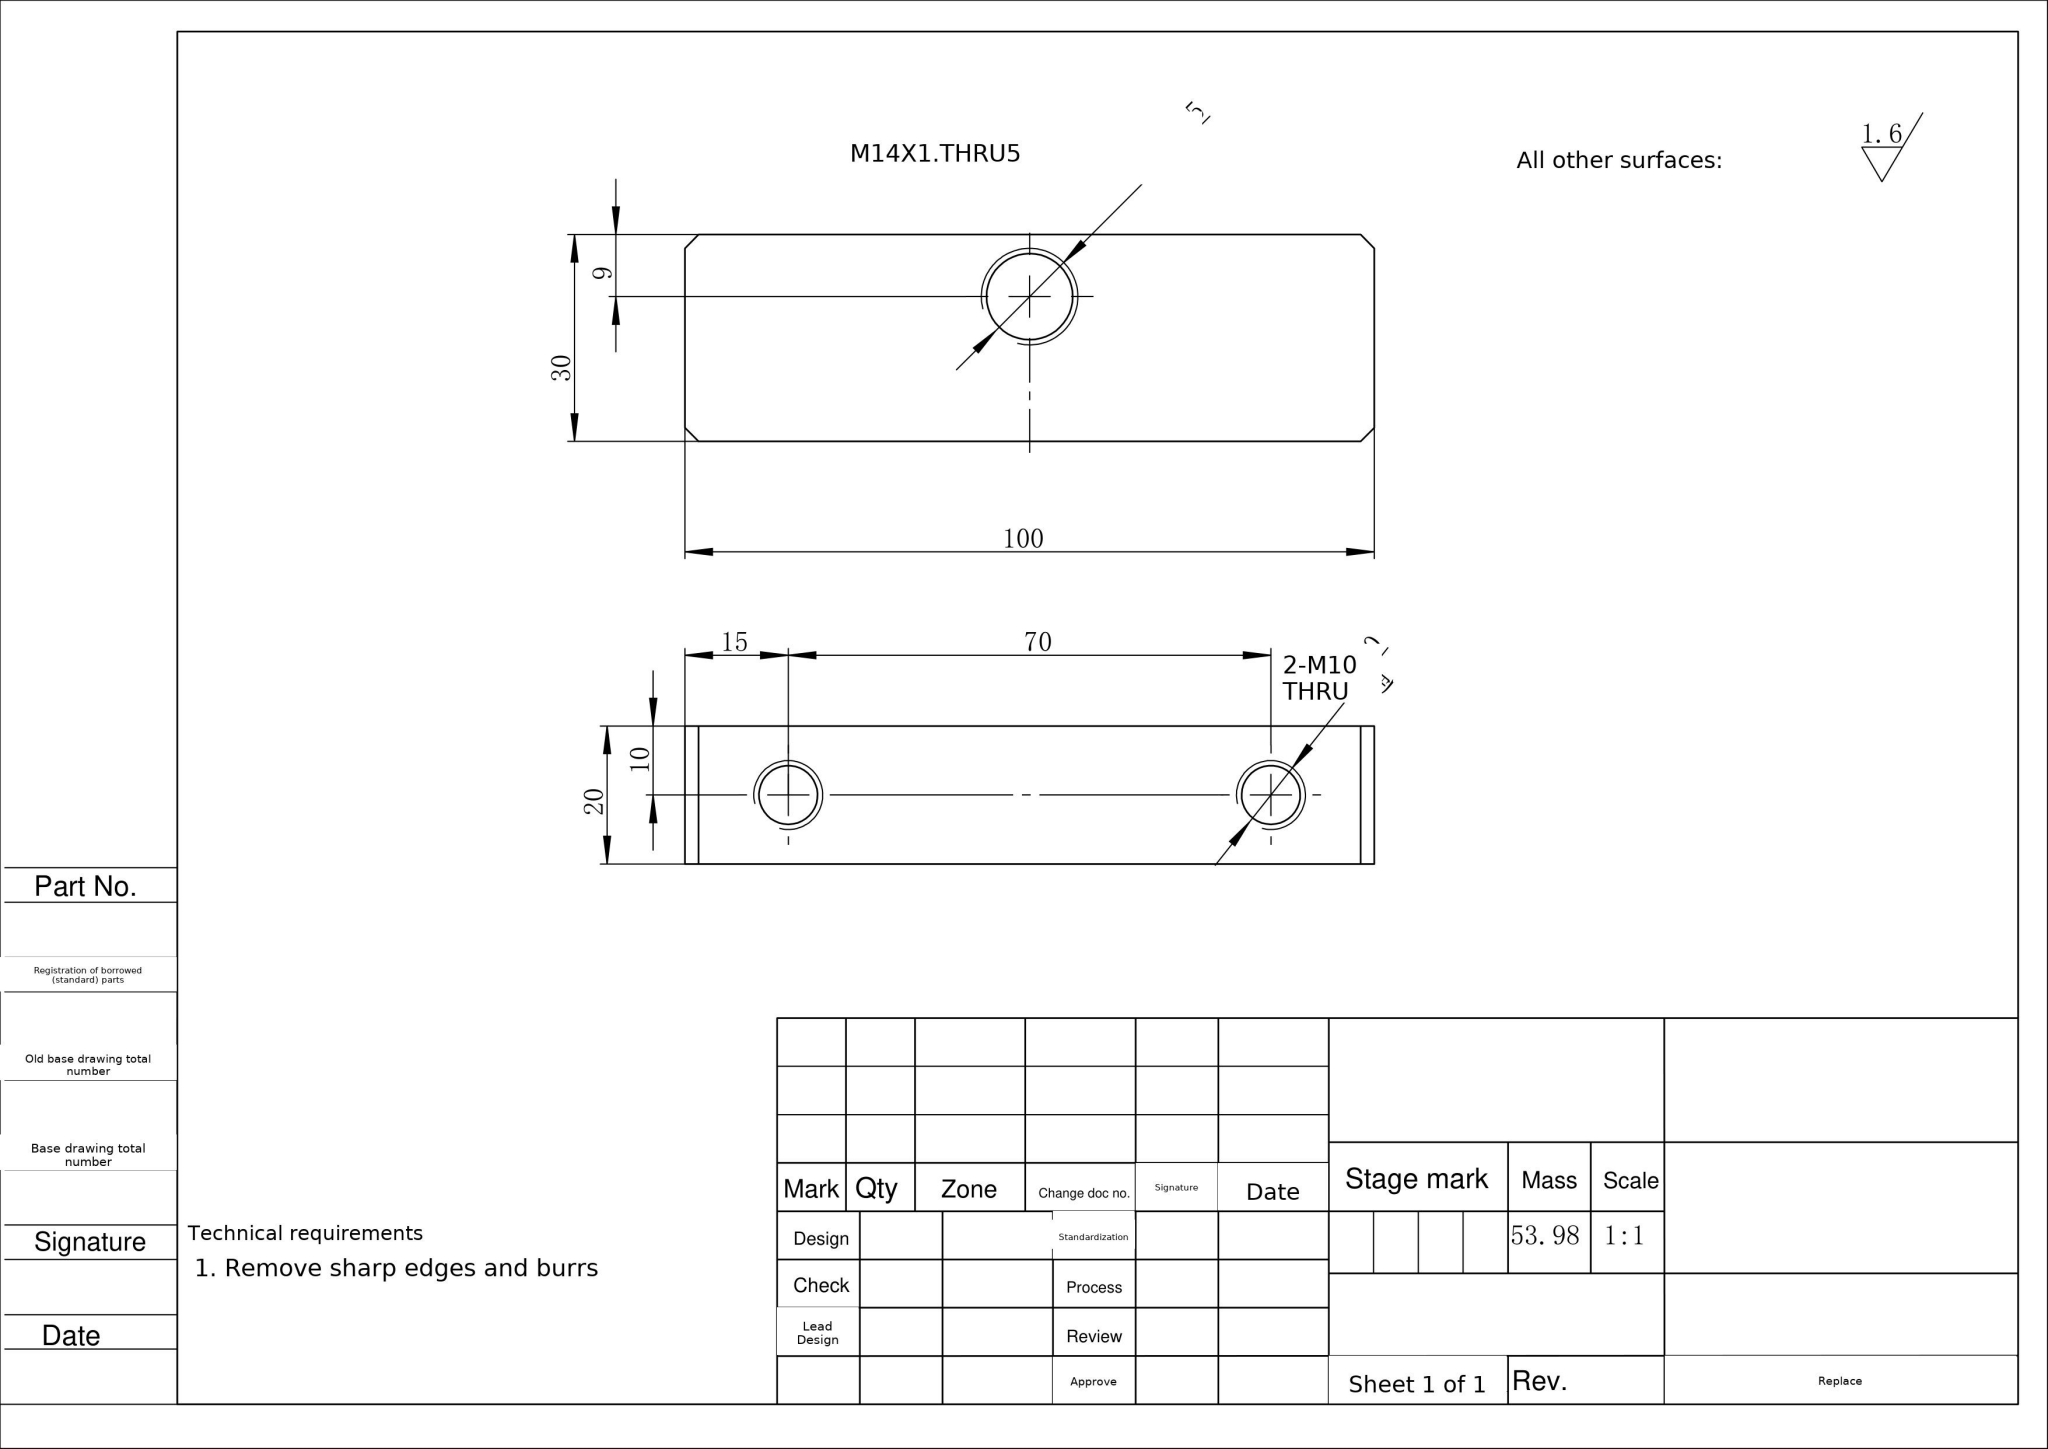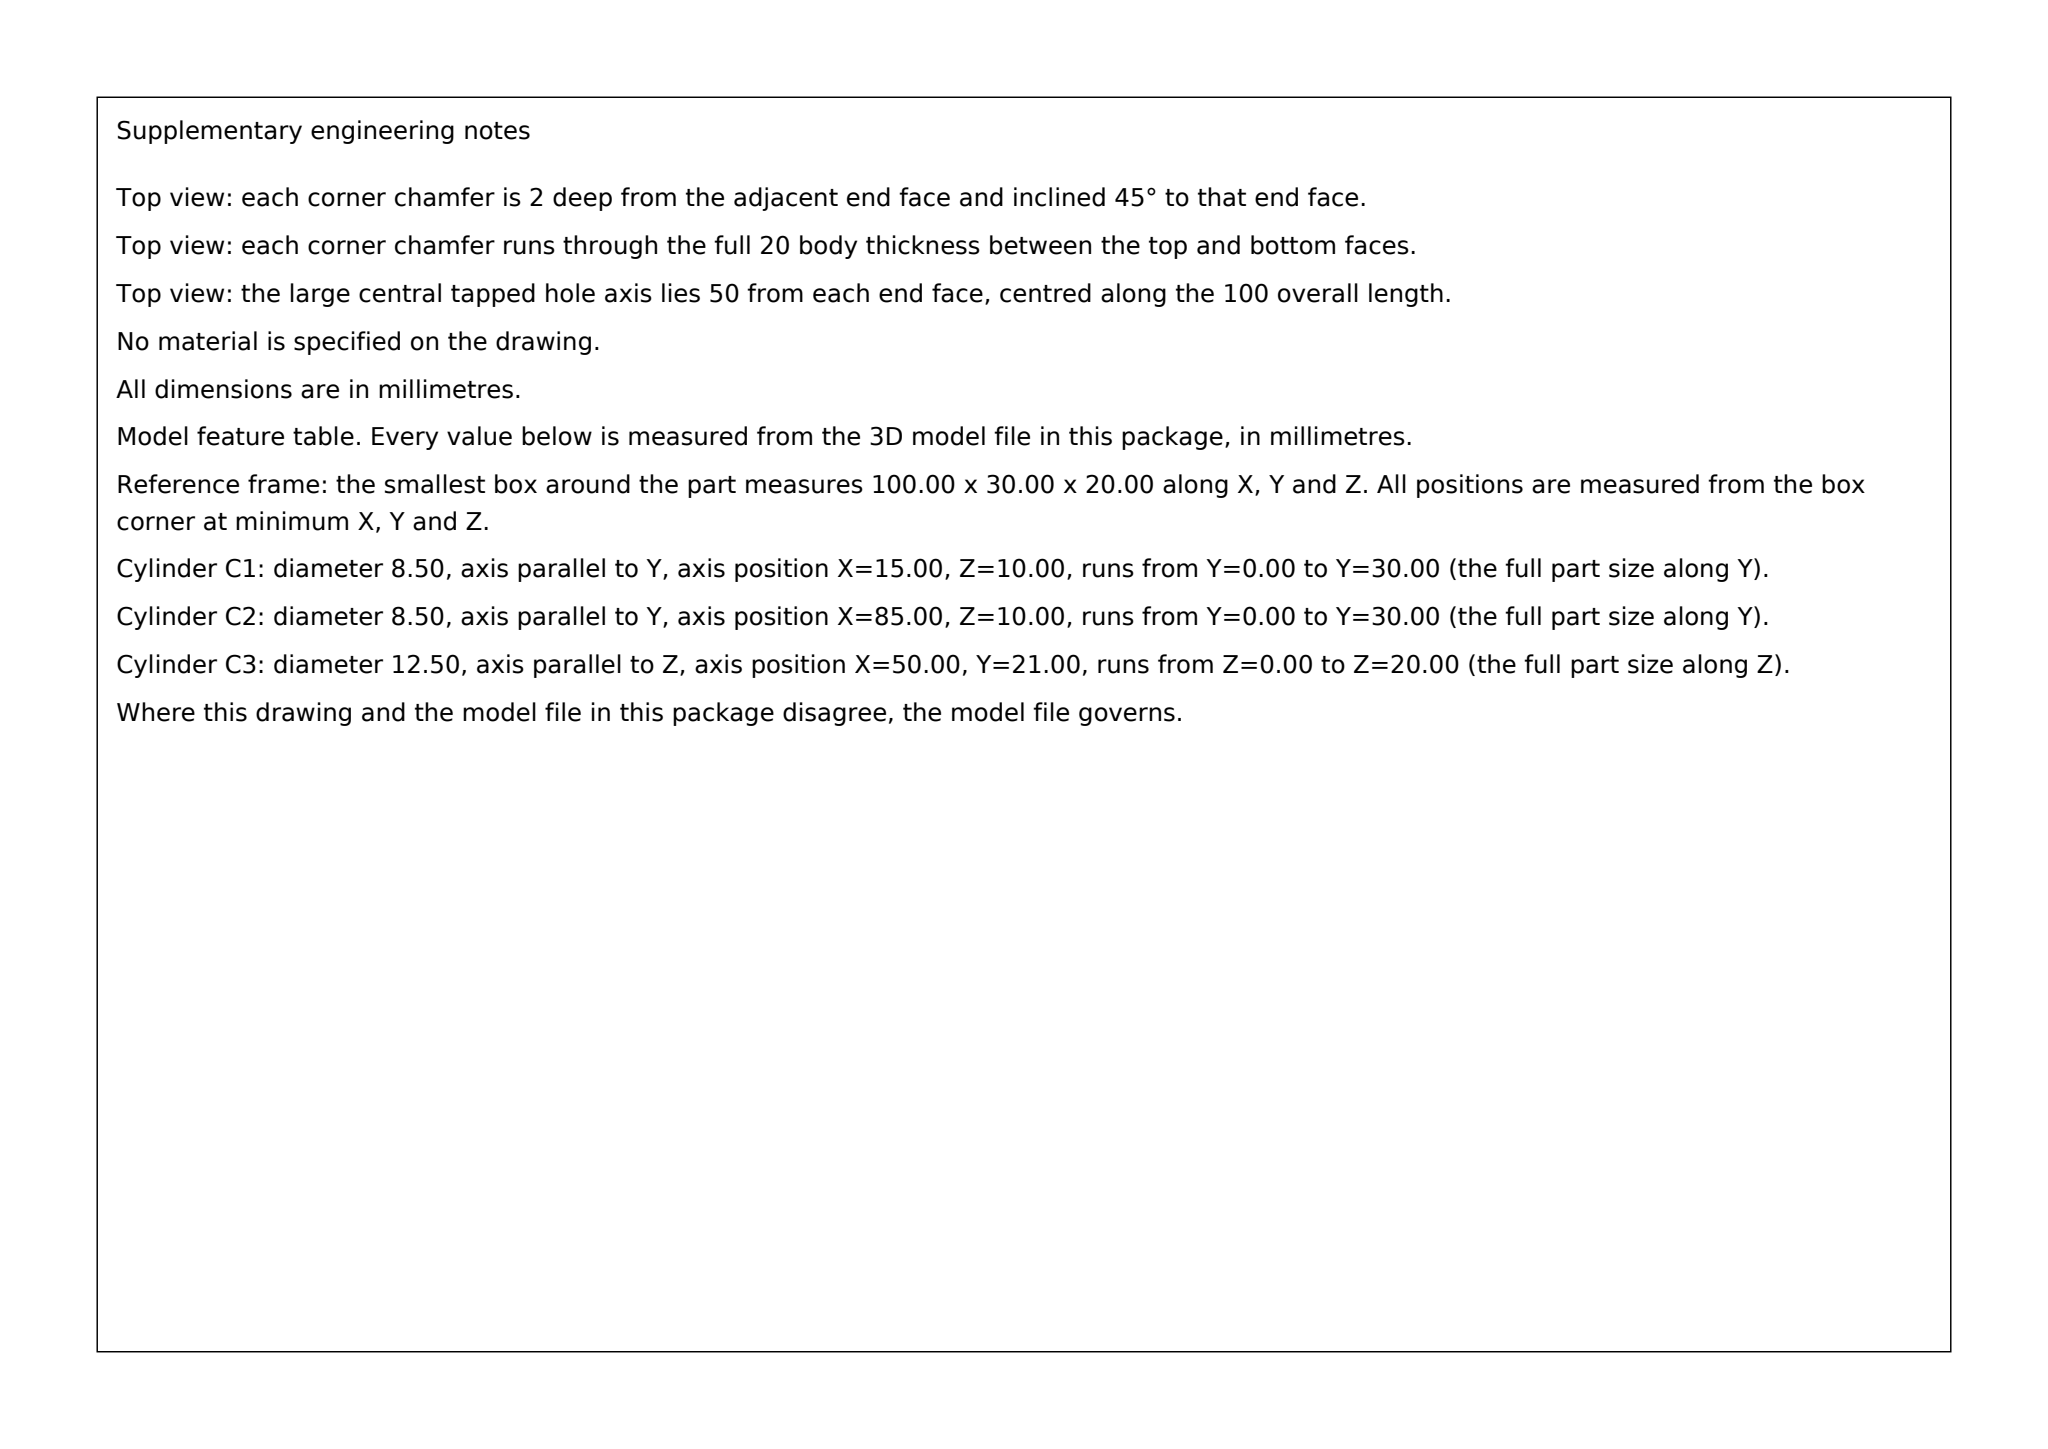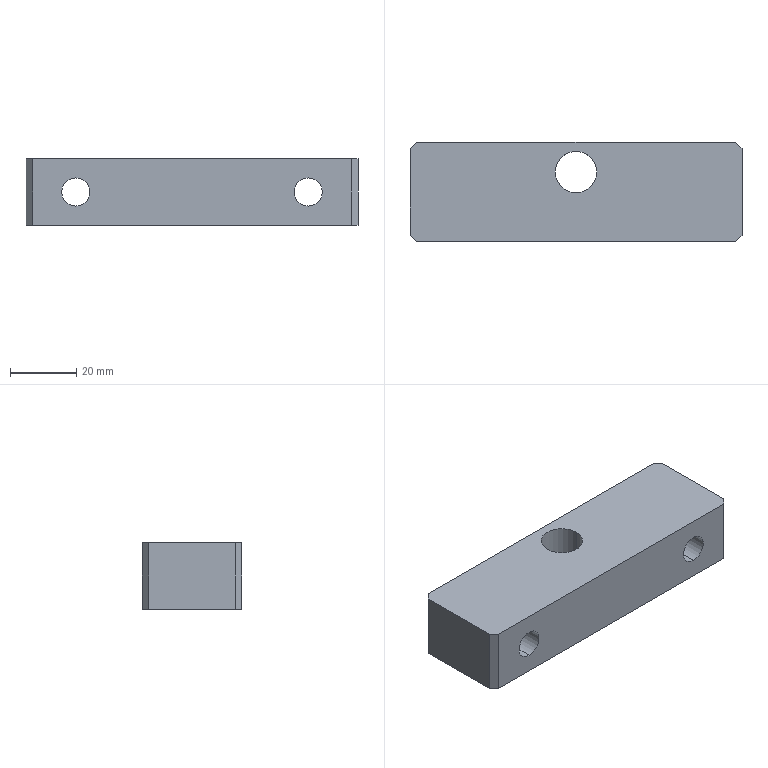Part | SolidWorks | mm | 1 solid | 16 faces | box 100 x 30 x 20 mm | volume 53981 mm3 | plane 10 | cylinder 6 | commonest cylinder face diameters 8.5 x4 12.5 x2
Drawing notes:
M14X1 THRU (THRU 20 THK) - NOT 5 DEEP | from the solid: cylinder dia 12.5, axis z, pos (50,21), length 20 = full 20 thk
M14X1 HOLE CL 50 FROM LEFT END, 9 FROM TOP EDGE | from the solid: cyl axis at x=50 of 100 bbox; y=21 of 30 -> 9 from top face y=30
build123d program:
from build123d import *

# Parameters (mm, degrees)
SKETCH1_W              = 100
SKETCH1_H              = 30
BOSS_EXTRUDE1_DEPTH    = 20
M10_TAPPED_HOLE1_D     = 8.5
M14X1_5_TAPPED_HOLE1_D = 12.5
CHAMFER1_SIZE          = 2


with BuildPart() as part:
    # Sketch1 → Boss-Extrude1 (new body)
    with BuildSketch(Plane.XY):
        Rectangle(SKETCH1_W, SKETCH1_H)
    extrude(amount=BOSS_EXTRUDE1_DEPTH)

    # M10 Tapped Hole1 (through all)
    with Locations(Plane(origin=(0, 15, 0), x_dir=(1, 0, 0), z_dir=(0, 1, 0))):
        with Locations((-35, -10), (35, -10)):
            Hole(M10_TAPPED_HOLE1_D / 2)

    # M14x1.5 Tapped Hole1 (through all)
    with Locations(Plane.XY.offset(20)):
        with Locations((0, 6)):
            Hole(M14X1_5_TAPPED_HOLE1_D / 2)

    # Chamfer1
    chamfer1_edges = [part.edges().sort_by_distance(p)[0] for p in [
        (50, -15, 10),
        (-50, -15, 10),
        (-50, 15, 10),
        (50, 15, 10),
    ]]
    chamfer(chamfer1_edges, length=CHAMFER1_SIZE)


solid = part.part
STEP:
#1=CARTESIAN_POINT('',(6.25,6.,0.));
#2=VERTEX_POINT('',#1);
#3=CARTESIAN_POINT('',(-6.25,6.,0.));
#4=VERTEX_POINT('',#3);
#5=CARTESIAN_POINT('',(0.,6.,0.));
#6=DIRECTION('',(0.,0.,-1.));
#7=DIRECTION('',(-1.,0.,0.));
#8=AXIS2_PLACEMENT_3D('',#5,#6,#7);
#9=CIRCLE('',#8,6.25);
#10=EDGE_CURVE('',#2,#4,#9,.T.);
#11=ORIENTED_EDGE('',*,*,#10,.T.);
#12=CARTESIAN_POINT('',(-6.25,6.,20.));
#13=VERTEX_POINT('',#12);
#14=CARTESIAN_POINT('',(-6.25,6.,20.));
#15=DIRECTION('',(0.,0.,1.));
#16=VECTOR('',#15,1000.);
#17=LINE('',#14,#16);
#18=EDGE_CURVE('',#4,#13,#17,.T.);
#19=ORIENTED_EDGE('',*,*,#18,.T.);
#20=CARTESIAN_POINT('',(6.25,6.,20.));
#21=VERTEX_POINT('',#20);
#22=CARTESIAN_POINT('',(0.,6.,20.));
#23=DIRECTION('',(0.,0.,1.));
#24=DIRECTION('',(1.,0.,0.));
#25=AXIS2_PLACEMENT_3D('',#22,#23,#24);
#26=CIRCLE('',#25,6.25);
#27=EDGE_CURVE('',#13,#21,#26,.T.);
#28=ORIENTED_EDGE('',*,*,#27,.T.);
#29=CARTESIAN_POINT('',(6.25,6.,20.));
#30=DIRECTION('',(0.,0.,1.));
#31=VECTOR('',#30,1000.);
#32=LINE('',#29,#31);
#33=EDGE_CURVE('',#2,#21,#32,.T.);
#34=ORIENTED_EDGE('',*,*,#33,.F.);
#35=EDGE_LOOP('',(#11,#19,#28,#34));
#36=FACE_OUTER_BOUND('',#35,.T.);
#37=CARTESIAN_POINT('',(0.,6.,20.));
#38=DIRECTION('',(0.,0.,1.));
#39=DIRECTION('',(1.,0.,0.));
#40=AXIS2_PLACEMENT_3D('',#37,#38,#39);
#41=CYLINDRICAL_SURFACE('',#40,6.25);
#42=ADVANCED_FACE('',(#36),#41,.F.);
#43=CARTESIAN_POINT('',(-35.,-15.,5.75));
#44=VERTEX_POINT('',#43);
#45=CARTESIAN_POINT('',(-35.,-15.,14.25));
#46=VERTEX_POINT('',#45);
#47=CARTESIAN_POINT('',(-35.,-15.,10.));
#48=DIRECTION('',(0.,1.,0.));
#49=DIRECTION('',(0.,0.,1.));
#50=AXIS2_PLACEMENT_3D('',#47,#48,#49);
#51=CIRCLE('',#50,4.25);
#52=EDGE_CURVE('',#44,#46,#51,.T.);
#53=ORIENTED_EDGE('',*,*,#52,.F.);
#54=CARTESIAN_POINT('',(-35.,15.,5.75));
#55=VERTEX_POINT('',#54);
#56=CARTESIAN_POINT('',(-35.,15.,5.75));
#57=DIRECTION('',(0.,1.,0.));
#58=VECTOR('',#57,1000.);
#59=LINE('',#56,#58);
#60=EDGE_CURVE('',#44,#55,#59,.T.);
#61=ORIENTED_EDGE('',*,*,#60,.T.);
#62=CARTESIAN_POINT('',(-35.,15.,14.25));
#63=VERTEX_POINT('',#62);
#64=CARTESIAN_POINT('',(-35.,15.,10.));
#65=DIRECTION('',(0.,1.,0.));
#66=DIRECTION('',(0.,0.,1.));
#67=AXIS2_PLACEMENT_3D('',#64,#65,#66);
#68=CIRCLE('',#67,4.25);
#69=EDGE_CURVE('',#55,#63,#68,.T.);
#70=ORIENTED_EDGE('',*,*,#69,.T.);
#71=CARTESIAN_POINT('',(-35.,15.,14.25));
#72=DIRECTION('',(0.,1.,0.));
#73=VECTOR('',#72,1000.);
#74=LINE('',#71,#73);
#75=EDGE_CURVE('',#46,#63,#74,.T.);
#76=ORIENTED_EDGE('',*,*,#75,.F.);
#77=EDGE_LOOP('',(#53,#61,#70,#76));
#78=FACE_OUTER_BOUND('',#77,.T.);
#79=CARTESIAN_POINT('',(-35.,15.,10.));
#80=DIRECTION('',(0.,1.,0.));
#81=DIRECTION('',(0.,0.,1.));
#82=AXIS2_PLACEMENT_3D('',#79,#80,#81);
#83=CYLINDRICAL_SURFACE('',#82,4.25);
#84=ADVANCED_FACE('',(#78),#83,.F.);
#85=CARTESIAN_POINT('',(35.,-15.,5.75));
#86=VERTEX_POINT('',#85);
#87=CARTESIAN_POINT('',(35.,-15.,14.25));
#88=VERTEX_POINT('',#87);
#89=CARTESIAN_POINT('',(35.,-15.,10.));
#90=DIRECTION('',(0.,1.,0.));
#91=DIRECTION('',(0.,0.,1.));
#92=AXIS2_PLACEMENT_3D('',#89,#90,#91);
#93=CIRCLE('',#92,4.25);
#94=EDGE_CURVE('',#86,#88,#93,.T.);
#95=ORIENTED_EDGE('',*,*,#94,.F.);
#96=CARTESIAN_POINT('',(35.,15.,5.75));
#97=VERTEX_POINT('',#96);
#98=CARTESIAN_POINT('',(35.,15.,5.75));
#99=DIRECTION('',(0.,1.,0.));
#100=VECTOR('',#99,1000.);
#101=LINE('',#98,#100);
#102=EDGE_CURVE('',#86,#97,#101,.T.);
#103=ORIENTED_EDGE('',*,*,#102,.T.);
#104=CARTESIAN_POINT('',(35.,15.,14.25));
#105=VERTEX_POINT('',#104);
#106=CARTESIAN_POINT('',(35.,15.,10.));
#107=DIRECTION('',(0.,1.,0.));
#108=DIRECTION('',(0.,0.,1.));
#109=AXIS2_PLACEMENT_3D('',#106,#107,#108);
#110=CIRCLE('',#109,4.25);
#111=EDGE_CURVE('',#97,#105,#110,.T.);
#112=ORIENTED_EDGE('',*,*,#111,.T.);
#113=CARTESIAN_POINT('',(35.,15.,14.25));
#114=DIRECTION('',(0.,1.,0.));
#115=VECTOR('',#114,1000.);
#116=LINE('',#113,#115);
#117=EDGE_CURVE('',#88,#105,#116,.T.);
#118=ORIENTED_EDGE('',*,*,#117,.F.);
#119=EDGE_LOOP('',(#95,#103,#112,#118));
#120=FACE_OUTER_BOUND('',#119,.T.);
#121=CARTESIAN_POINT('',(35.,15.,10.));
#122=DIRECTION('',(0.,1.,0.));
#123=DIRECTION('',(0.,0.,1.));
#124=AXIS2_PLACEMENT_3D('',#121,#122,#123);
#125=CYLINDRICAL_SURFACE('',#124,4.25);
#126=ADVANCED_FACE('',(#120),#125,.F.);
#127=CARTESIAN_POINT('',(48.,15.,0.));
#128=VERTEX_POINT('',#127);
#129=CARTESIAN_POINT('',(-48.,15.,0.));
#130=VERTEX_POINT('',#129);
#131=CARTESIAN_POINT('',(-50.,15.,0.));
#132=DIRECTION('',(-1.,0.,0.));
#133=VECTOR('',#132,1000.);
#134=LINE('',#131,#133);
#135=EDGE_CURVE('',#128,#130,#134,.T.);
#136=ORIENTED_EDGE('',*,*,#135,.T.);
#137=CARTESIAN_POINT('',(-48.,15.,20.));
#138=VERTEX_POINT('',#137);
#139=CARTESIAN_POINT('',(-48.,15.,20.));
#140=DIRECTION('',(0.,0.,1.));
#141=VECTOR('',#140,1000.);
#142=LINE('',#139,#141);
#143=EDGE_CURVE('',#130,#138,#142,.T.);
#144=ORIENTED_EDGE('',*,*,#143,.T.);
#145=CARTESIAN_POINT('',(48.,15.,20.));
#146=VERTEX_POINT('',#145);
#147=CARTESIAN_POINT('',(-50.,15.,20.));
#148=DIRECTION('',(-1.,0.,0.));
#149=VECTOR('',#148,1000.);
#150=LINE('',#147,#149);
#151=EDGE_CURVE('',#146,#138,#150,.T.);
#152=ORIENTED_EDGE('',*,*,#151,.F.);
#153=CARTESIAN_POINT('',(48.,15.,20.));
#154=DIRECTION('',(0.,0.,-1.));
#155=VECTOR('',#154,1000.);
#156=LINE('',#153,#155);
#157=EDGE_CURVE('',#146,#128,#156,.T.);
#158=ORIENTED_EDGE('',*,*,#157,.T.);
#159=EDGE_LOOP('',(#136,#144,#152,#158));
#160=FACE_OUTER_BOUND('',#159,.T.);
#161=CARTESIAN_POINT('',(35.,15.,10.));
#162=DIRECTION('',(0.,1.,0.));
#163=DIRECTION('',(0.,0.,1.));
#164=AXIS2_PLACEMENT_3D('',#161,#162,#163);
#165=CIRCLE('',#164,4.25);
#166=EDGE_CURVE('',#105,#97,#165,.T.);
#167=ORIENTED_EDGE('',*,*,#166,.F.);
#168=ORIENTED_EDGE('',*,*,#111,.F.);
#169=EDGE_LOOP('',(#167,#168));
#170=FACE_BOUND('',#169,.T.);
#171=CARTESIAN_POINT('',(-35.,15.,10.));
#172=DIRECTION('',(0.,1.,0.));
#173=DIRECTION('',(0.,0.,1.));
#174=AXIS2_PLACEMENT_3D('',#171,#172,#173);
#175=CIRCLE('',#174,4.25);
#176=EDGE_CURVE('',#63,#55,#175,.T.);
#177=ORIENTED_EDGE('',*,*,#176,.F.);
#178=ORIENTED_EDGE('',*,*,#69,.F.);
#179=EDGE_LOOP('',(#177,#178));
#180=FACE_BOUND('',#179,.T.);
#181=CARTESIAN_POINT('',(-50.,15.,20.));
#182=DIRECTION('',(0.,-1.,0.));
#183=DIRECTION('',(0.,0.,-1.));
#184=AXIS2_PLACEMENT_3D('',#181,#182,#183);
#185=PLANE('',#184);
#186=ADVANCED_FACE('',(#160,#170,#180),#185,.F.);
#187=CARTESIAN_POINT('',(50.,-13.,0.));
#188=VERTEX_POINT('',#187);
#189=CARTESIAN_POINT('',(50.,13.,0.));
#190=VERTEX_POINT('',#189);
#191=CARTESIAN_POINT('',(50.,-15.,0.));
#192=DIRECTION('',(0.,1.,0.));
#193=VECTOR('',#192,1000.);
#194=LINE('',#191,#193);
#195=EDGE_CURVE('',#188,#190,#194,.T.);
#196=ORIENTED_EDGE('',*,*,#195,.T.);
#197=CARTESIAN_POINT('',(50.,13.,20.));
#198=VERTEX_POINT('',#197);
#199=CARTESIAN_POINT('',(50.,13.,20.));
#200=DIRECTION('',(0.,0.,1.));
#201=VECTOR('',#200,1000.);
#202=LINE('',#199,#201);
#203=EDGE_CURVE('',#190,#198,#202,.T.);
#204=ORIENTED_EDGE('',*,*,#203,.T.);
#205=CARTESIAN_POINT('',(50.,-13.,20.));
#206=VERTEX_POINT('',#205);
#207=CARTESIAN_POINT('',(50.,-15.,20.));
#208=DIRECTION('',(0.,1.,0.));
#209=VECTOR('',#208,1000.);
#210=LINE('',#207,#209);
#211=EDGE_CURVE('',#206,#198,#210,.T.);
#212=ORIENTED_EDGE('',*,*,#211,.F.);
#213=CARTESIAN_POINT('',(50.,-13.,20.));
#214=DIRECTION('',(0.,0.,-1.));
#215=VECTOR('',#214,1000.);
#216=LINE('',#213,#215);
#217=EDGE_CURVE('',#206,#188,#216,.T.);
#218=ORIENTED_EDGE('',*,*,#217,.T.);
#219=EDGE_LOOP('',(#196,#204,#212,#218));
#220=FACE_OUTER_BOUND('',#219,.T.);
#221=CARTESIAN_POINT('',(50.,-15.,20.));
#222=DIRECTION('',(-1.,0.,0.));
#223=DIRECTION('',(0.,0.,1.));
#224=AXIS2_PLACEMENT_3D('',#221,#222,#223);
#225=PLANE('',#224);
#226=ADVANCED_FACE('',(#220),#225,.F.);
#227=CARTESIAN_POINT('',(-50.,13.,0.));
#228=VERTEX_POINT('',#227);
#229=CARTESIAN_POINT('',(-50.,-13.,0.));
#230=VERTEX_POINT('',#229);
#231=CARTESIAN_POINT('',(-50.,-15.,0.));
#232=DIRECTION('',(0.,-1.,0.));
#233=VECTOR('',#232,1000.);
#234=LINE('',#231,#233);
#235=EDGE_CURVE('',#228,#230,#234,.T.);
#236=ORIENTED_EDGE('',*,*,#235,.T.);
#237=CARTESIAN_POINT('',(-50.,-13.,20.));
#238=VERTEX_POINT('',#237);
#239=CARTESIAN_POINT('',(-50.,-13.,20.));
#240=DIRECTION('',(0.,0.,1.));
#241=VECTOR('',#240,1000.);
#242=LINE('',#239,#241);
#243=EDGE_CURVE('',#230,#238,#242,.T.);
#244=ORIENTED_EDGE('',*,*,#243,.T.);
#245=CARTESIAN_POINT('',(-50.,13.,20.));
#246=VERTEX_POINT('',#245);
#247=CARTESIAN_POINT('',(-50.,-15.,20.));
#248=DIRECTION('',(0.,-1.,0.));
#249=VECTOR('',#248,1000.);
#250=LINE('',#247,#249);
#251=EDGE_CURVE('',#246,#238,#250,.T.);
#252=ORIENTED_EDGE('',*,*,#251,.F.);
#253=CARTESIAN_POINT('',(-50.,13.,20.));
#254=DIRECTION('',(0.,0.,-1.));
#255=VECTOR('',#254,1000.);
#256=LINE('',#253,#255);
#257=EDGE_CURVE('',#246,#228,#256,.T.);
#258=ORIENTED_EDGE('',*,*,#257,.T.);
#259=EDGE_LOOP('',(#236,#244,#252,#258));
#260=FACE_OUTER_BOUND('',#259,.T.);
#261=CARTESIAN_POINT('',(-50.,-15.,20.));
#262=DIRECTION('',(1.,0.,0.));
#263=DIRECTION('',(0.,0.,-1.));
#264=AXIS2_PLACEMENT_3D('',#261,#262,#263);
#265=PLANE('',#264);
#266=ADVANCED_FACE('',(#260),#265,.F.);
#267=CARTESIAN_POINT('',(-35.,-15.,10.));
#268=DIRECTION('',(0.,1.,0.));
#269=DIRECTION('',(0.,0.,1.));
#270=AXIS2_PLACEMENT_3D('',#267,#268,#269);
#271=CIRCLE('',#270,4.25);
#272=EDGE_CURVE('',#46,#44,#271,.T.);
#273=ORIENTED_EDGE('',*,*,#272,.T.);
#274=ORIENTED_EDGE('',*,*,#52,.T.);
#275=EDGE_LOOP('',(#273,#274));
#276=FACE_BOUND('',#275,.T.);
#277=CARTESIAN_POINT('',(35.,-15.,10.));
#278=DIRECTION('',(0.,1.,0.));
#279=DIRECTION('',(0.,0.,1.));
#280=AXIS2_PLACEMENT_3D('',#277,#278,#279);
#281=CIRCLE('',#280,4.25);
#282=EDGE_CURVE('',#88,#86,#281,.T.);
#283=ORIENTED_EDGE('',*,*,#282,.T.);
#284=ORIENTED_EDGE('',*,*,#94,.T.);
#285=EDGE_LOOP('',(#283,#284));
#286=FACE_BOUND('',#285,.T.);
#287=CARTESIAN_POINT('',(-48.,-15.,20.));
#288=VERTEX_POINT('',#287);
#289=CARTESIAN_POINT('',(48.,-15.,20.));
#290=VERTEX_POINT('',#289);
#291=CARTESIAN_POINT('',(-50.,-15.,20.));
#292=DIRECTION('',(1.,0.,0.));
#293=VECTOR('',#292,1000.);
#294=LINE('',#291,#293);
#295=EDGE_CURVE('',#288,#290,#294,.T.);
#296=ORIENTED_EDGE('',*,*,#295,.F.);
#297=CARTESIAN_POINT('',(-48.,-15.,0.));
#298=VERTEX_POINT('',#297);
#299=CARTESIAN_POINT('',(-48.,-15.,20.));
#300=DIRECTION('',(0.,0.,-1.));
#301=VECTOR('',#300,1000.);
#302=LINE('',#299,#301);
#303=EDGE_CURVE('',#288,#298,#302,.T.);
#304=ORIENTED_EDGE('',*,*,#303,.T.);
#305=CARTESIAN_POINT('',(48.,-15.,0.));
#306=VERTEX_POINT('',#305);
#307=CARTESIAN_POINT('',(-50.,-15.,0.));
#308=DIRECTION('',(1.,0.,0.));
#309=VECTOR('',#308,1000.);
#310=LINE('',#307,#309);
#311=EDGE_CURVE('',#298,#306,#310,.T.);
#312=ORIENTED_EDGE('',*,*,#311,.T.);
#313=CARTESIAN_POINT('',(48.,-15.,20.));
#314=DIRECTION('',(0.,0.,1.));
#315=VECTOR('',#314,1000.);
#316=LINE('',#313,#315);
#317=EDGE_CURVE('',#306,#290,#316,.T.);
#318=ORIENTED_EDGE('',*,*,#317,.T.);
#319=EDGE_LOOP('',(#296,#304,#312,#318));
#320=FACE_OUTER_BOUND('',#319,.T.);
#321=CARTESIAN_POINT('',(-50.,-15.,20.));
#322=DIRECTION('',(0.,1.,0.));
#323=DIRECTION('',(0.,0.,1.));
#324=AXIS2_PLACEMENT_3D('',#321,#322,#323);
#325=PLANE('',#324);
#326=ADVANCED_FACE('',(#276,#286,#320),#325,.F.);
#327=CARTESIAN_POINT('',(0.,6.,20.));
#328=DIRECTION('',(0.,0.,1.));
#329=DIRECTION('',(1.,0.,0.));
#330=AXIS2_PLACEMENT_3D('',#327,#328,#329);
#331=CIRCLE('',#330,6.25);
#332=EDGE_CURVE('',#21,#13,#331,.T.);
#333=ORIENTED_EDGE('',*,*,#332,.F.);
#334=ORIENTED_EDGE('',*,*,#27,.F.);
#335=EDGE_LOOP('',(#333,#334));
#336=FACE_BOUND('',#335,.T.);
#337=ORIENTED_EDGE('',*,*,#251,.T.);
#338=CARTESIAN_POINT('',(-48.,-15.,20.));
#339=DIRECTION('',(0.7071,-0.7071,0.));
#340=VECTOR('',#339,1000.);
#341=LINE('',#338,#340);
#342=EDGE_CURVE('',#238,#288,#341,.T.);
#343=ORIENTED_EDGE('',*,*,#342,.T.);
#344=ORIENTED_EDGE('',*,*,#295,.T.);
#345=CARTESIAN_POINT('',(50.,-13.,20.));
#346=DIRECTION('',(0.7071,0.7071,0.));
#347=VECTOR('',#346,1000.);
#348=LINE('',#345,#347);
#349=EDGE_CURVE('',#290,#206,#348,.T.);
#350=ORIENTED_EDGE('',*,*,#349,.T.);
#351=ORIENTED_EDGE('',*,*,#211,.T.);
#352=CARTESIAN_POINT('',(48.,15.,20.));
#353=DIRECTION('',(-0.7071,0.7071,0.));
#354=VECTOR('',#353,1000.);
#355=LINE('',#352,#354);
#356=EDGE_CURVE('',#198,#146,#355,.T.);
#357=ORIENTED_EDGE('',*,*,#356,.T.);
#358=ORIENTED_EDGE('',*,*,#151,.T.);
#359=CARTESIAN_POINT('',(-50.,13.,20.));
#360=DIRECTION('',(-0.7071,-0.7071,0.));
#361=VECTOR('',#360,1000.);
#362=LINE('',#359,#361);
#363=EDGE_CURVE('',#138,#246,#362,.T.);
#364=ORIENTED_EDGE('',*,*,#363,.T.);
#365=EDGE_LOOP('',(#337,#343,#344,#350,#351,#357,#358,#364));
#366=FACE_OUTER_BOUND('',#365,.T.);
#367=CARTESIAN_POINT('',(0.,0.,20.));
#368=DIRECTION('',(0.,0.,-1.));
#369=DIRECTION('',(-1.,0.,0.));
#370=AXIS2_PLACEMENT_3D('',#367,#368,#369);
#371=PLANE('',#370);
#372=ADVANCED_FACE('',(#336,#366),#371,.F.);
#373=ORIENTED_EDGE('',*,*,#10,.F.);
#374=CARTESIAN_POINT('',(0.,6.,0.));
#375=DIRECTION('',(0.,0.,-1.));
#376=DIRECTION('',(-1.,0.,0.));
#377=AXIS2_PLACEMENT_3D('',#374,#375,#376);
#378=CIRCLE('',#377,6.25);
#379=EDGE_CURVE('',#4,#2,#378,.T.);
#380=ORIENTED_EDGE('',*,*,#379,.F.);
#381=EDGE_LOOP('',(#373,#380));
#382=FACE_BOUND('',#381,.T.);
#383=ORIENTED_EDGE('',*,*,#311,.F.);
#384=CARTESIAN_POINT('',(-31.5,-31.5,0.));
#385=DIRECTION('',(-0.7071,0.7071,0.));
#386=VECTOR('',#385,1000.);
#387=LINE('',#384,#386);
#388=EDGE_CURVE('',#298,#230,#387,.T.);
#389=ORIENTED_EDGE('',*,*,#388,.T.);
#390=ORIENTED_EDGE('',*,*,#235,.F.);
#391=CARTESIAN_POINT('',(-31.5,31.5,0.));
#392=DIRECTION('',(0.7071,0.7071,0.));
#393=VECTOR('',#392,1000.);
#394=LINE('',#391,#393);
#395=EDGE_CURVE('',#228,#130,#394,.T.);
#396=ORIENTED_EDGE('',*,*,#395,.T.);
#397=ORIENTED_EDGE('',*,*,#135,.F.);
#398=CARTESIAN_POINT('',(31.5,31.5,0.));
#399=DIRECTION('',(0.7071,-0.7071,0.));
#400=VECTOR('',#399,1000.);
#401=LINE('',#398,#400);
#402=EDGE_CURVE('',#128,#190,#401,.T.);
#403=ORIENTED_EDGE('',*,*,#402,.T.);
#404=ORIENTED_EDGE('',*,*,#195,.F.);
#405=CARTESIAN_POINT('',(31.5,-31.5,0.));
#406=DIRECTION('',(-0.7071,-0.7071,0.));
#407=VECTOR('',#406,1000.);
#408=LINE('',#405,#407);
#409=EDGE_CURVE('',#188,#306,#408,.T.);
#410=ORIENTED_EDGE('',*,*,#409,.T.);
#411=EDGE_LOOP('',(#383,#389,#390,#396,#397,#403,#404,#410));
#412=FACE_OUTER_BOUND('',#411,.T.);
#413=CARTESIAN_POINT('',(0.,0.,0.));
#414=DIRECTION('',(0.,0.,-1.));
#415=DIRECTION('',(-1.,0.,0.));
#416=AXIS2_PLACEMENT_3D('',#413,#414,#415);
#417=PLANE('',#416);
#418=ADVANCED_FACE('',(#382,#412),#417,.T.);
#419=ORIENTED_EDGE('',*,*,#102,.F.);
#420=ORIENTED_EDGE('',*,*,#282,.F.);
#421=ORIENTED_EDGE('',*,*,#117,.T.);
#422=ORIENTED_EDGE('',*,*,#166,.T.);
#423=EDGE_LOOP('',(#419,#420,#421,#422));
#424=FACE_OUTER_BOUND('',#423,.T.);
#425=CARTESIAN_POINT('',(35.,15.,10.));
#426=DIRECTION('',(0.,1.,0.));
#427=DIRECTION('',(0.,0.,1.));
#428=AXIS2_PLACEMENT_3D('',#425,#426,#427);
#429=CYLINDRICAL_SURFACE('',#428,4.25);
#430=ADVANCED_FACE('',(#424),#429,.F.);
#431=ORIENTED_EDGE('',*,*,#60,.F.);
#432=ORIENTED_EDGE('',*,*,#272,.F.);
#433=ORIENTED_EDGE('',*,*,#75,.T.);
#434=ORIENTED_EDGE('',*,*,#176,.T.);
#435=EDGE_LOOP('',(#431,#432,#433,#434));
#436=FACE_OUTER_BOUND('',#435,.T.);
#437=CARTESIAN_POINT('',(-35.,15.,10.));
#438=DIRECTION('',(0.,1.,0.));
#439=DIRECTION('',(0.,0.,1.));
#440=AXIS2_PLACEMENT_3D('',#437,#438,#439);
#441=CYLINDRICAL_SURFACE('',#440,4.25);
#442=ADVANCED_FACE('',(#436),#441,.F.);
#443=ORIENTED_EDGE('',*,*,#18,.F.);
#444=ORIENTED_EDGE('',*,*,#379,.T.);
#445=ORIENTED_EDGE('',*,*,#33,.T.);
#446=ORIENTED_EDGE('',*,*,#332,.T.);
#447=EDGE_LOOP('',(#443,#444,#445,#446));
#448=FACE_OUTER_BOUND('',#447,.T.);
#449=CARTESIAN_POINT('',(0.,6.,20.));
#450=DIRECTION('',(0.,0.,1.));
#451=DIRECTION('',(1.,0.,0.));
#452=AXIS2_PLACEMENT_3D('',#449,#450,#451);
#453=CYLINDRICAL_SURFACE('',#452,6.25);
#454=ADVANCED_FACE('',(#448),#453,.F.);
#455=ORIENTED_EDGE('',*,*,#342,.F.);
#456=ORIENTED_EDGE('',*,*,#243,.F.);
#457=ORIENTED_EDGE('',*,*,#388,.F.);
#458=ORIENTED_EDGE('',*,*,#303,.F.);
#459=EDGE_LOOP('',(#455,#456,#457,#458));
#460=FACE_OUTER_BOUND('',#459,.T.);
#461=CARTESIAN_POINT('',(-48.,-15.,20.));
#462=DIRECTION('',(0.7071,0.7071,0.));
#463=DIRECTION('',(0.,0.,-1.));
#464=AXIS2_PLACEMENT_3D('',#461,#462,#463);
#465=PLANE('',#464);
#466=ADVANCED_FACE('',(#460),#465,.F.);
#467=ORIENTED_EDGE('',*,*,#363,.F.);
#468=ORIENTED_EDGE('',*,*,#143,.F.);
#469=ORIENTED_EDGE('',*,*,#395,.F.);
#470=ORIENTED_EDGE('',*,*,#257,.F.);
#471=EDGE_LOOP('',(#467,#468,#469,#470));
#472=FACE_OUTER_BOUND('',#471,.T.);
#473=CARTESIAN_POINT('',(-50.,13.,20.));
#474=DIRECTION('',(0.7071,-0.7071,0.));
#475=DIRECTION('',(0.,0.,-1.));
#476=AXIS2_PLACEMENT_3D('',#473,#474,#475);
#477=PLANE('',#476);
#478=ADVANCED_FACE('',(#472),#477,.F.);
#479=ORIENTED_EDGE('',*,*,#356,.F.);
#480=ORIENTED_EDGE('',*,*,#203,.F.);
#481=ORIENTED_EDGE('',*,*,#402,.F.);
#482=ORIENTED_EDGE('',*,*,#157,.F.);
#483=EDGE_LOOP('',(#479,#480,#481,#482));
#484=FACE_OUTER_BOUND('',#483,.T.);
#485=CARTESIAN_POINT('',(48.,15.,20.));
#486=DIRECTION('',(-0.7071,-0.7071,0.));
#487=DIRECTION('',(0.,0.,-1.));
#488=AXIS2_PLACEMENT_3D('',#485,#486,#487);
#489=PLANE('',#488);
#490=ADVANCED_FACE('',(#484),#489,.F.);
#491=ORIENTED_EDGE('',*,*,#349,.F.);
#492=ORIENTED_EDGE('',*,*,#317,.F.);
#493=ORIENTED_EDGE('',*,*,#409,.F.);
#494=ORIENTED_EDGE('',*,*,#217,.F.);
#495=EDGE_LOOP('',(#491,#492,#493,#494));
#496=FACE_OUTER_BOUND('',#495,.T.);
#497=CARTESIAN_POINT('',(50.,-13.,20.));
#498=DIRECTION('',(-0.7071,0.7071,0.));
#499=DIRECTION('',(0.,0.,-1.));
#500=AXIS2_PLACEMENT_3D('',#497,#498,#499);
#501=PLANE('',#500);
#502=ADVANCED_FACE('',(#496),#501,.F.);
#503=CLOSED_SHELL('',(#42,#84,#126,#186,#226,#266,#326,#372,#418,#430,#442,#454,#466,#478,#490,#502));
#504=MANIFOLD_SOLID_BREP('',#503);
#505=CARTESIAN_POINT('',(0.,0.,0.));
#506=DIRECTION('',(0.,0.,1.));
#507=DIRECTION('',(1.,0.,0.));
#508=AXIS2_PLACEMENT_3D('',#505,#506,#507);
#509=(LENGTH_UNIT()NAMED_UNIT(*)SI_UNIT(.MILLI.,.METRE.));
#510=UNCERTAINTY_MEASURE_WITH_UNIT(LENGTH_MEASURE(0.00001),#509,'','');
#511=(NAMED_UNIT(*)PLANE_ANGLE_UNIT()SI_UNIT($,.RADIAN.));
#512=(NAMED_UNIT(*)SI_UNIT($,.STERADIAN.)SOLID_ANGLE_UNIT());
#513=(GEOMETRIC_REPRESENTATION_CONTEXT(3)GLOBAL_UNCERTAINTY_ASSIGNED_CONTEXT((#510))GLOBAL_UNIT_ASSIGNED_CONTEXT((#509,#511,#512))REPRESENTATION_CONTEXT('',''));
#514=ADVANCED_BREP_SHAPE_REPRESENTATION('',(#504,#508),#513);